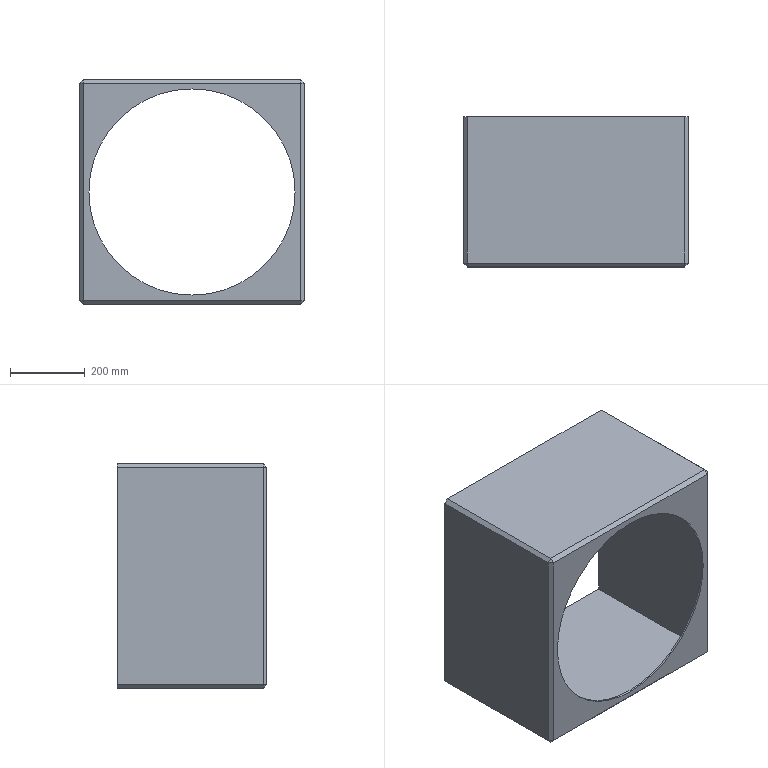Component | SolidWorks | Housing-1 | 1 solid | 25 faces | box 600 x 400 x 600 mm | volume 18742752 mm3 | plane 23 | cylinder 2 | commonest cylinder face diameters 550 x2
build123d program:
from build123d import *

# Parameters (mm, degrees)
SKETCH1_W           = 600
SKETCH1_H           = 600
SKETCH1_W_2         = 560
SKETCH1_H_2         = 560
BOSS_EXTRUDE1_DEPTH = 400
SKETCH2_W           = 560
SKETCH2_H           = 560
SKETCH2_R           = 275
BOSS_EXTRUDE2_DEPTH = 5
CHAMFER3_SIZE       = 10


with BuildPart() as part:
    # Sketch1 → Boss-Extrude1 (new body)
    with BuildSketch(Plane.XY):
        with Locations((-0.7059, 193.51)):
            Rectangle(SKETCH1_W, SKETCH1_H)
        with Locations((-0.7059, 193.51)):
            Rectangle(SKETCH1_W_2, SKETCH1_H_2, mode=Mode.SUBTRACT)
    extrude(amount=BOSS_EXTRUDE1_DEPTH)

    # Sketch2 → Boss-Extrude2 (add)
    with BuildSketch(Plane.XY.offset(400)):
        with Locations((-0.7059, 193.51)):
            Rectangle(SKETCH2_W, SKETCH2_H)
        with Locations((-0.7059, 193.51)):
            Circle(SKETCH2_R, mode=Mode.SUBTRACT)
    extrude(amount=-BOSS_EXTRUDE2_DEPTH)

    # Chamfer3
    chamfer3_edges = [part.edges().sort_by_distance(p)[0] for p in [
        (299.294, 193.51, 400),
        (-0.7059, 493.51, 400),
        (-300.706, 193.51, 400),
        (-300.706, 493.51, 200),
        (299.294, 493.51, 200),
        (299.294, -106.49, 200),
        (-300.706, -106.49, 200),
        (-0.7059, -106.49, 400),
    ]]
    chamfer(chamfer3_edges, length=CHAMFER3_SIZE)


solid = part.part

# Placed as in the assembly
solid = solid.moved(Location((0.7059, -200, -493.51), (90, 0, 0)))
STEP:
#1=COLOUR_RGB('',0.7922,0.8196,0.9333);
#2=FILL_AREA_STYLE_COLOUR('',#1);
#3=FILL_AREA_STYLE('',(#2));
#4=SURFACE_STYLE_FILL_AREA(#3);
#5=SURFACE_SIDE_STYLE('',(#4));
#6=SURFACE_STYLE_USAGE(.BOTH.,#5);
#7=PRESENTATION_STYLE_ASSIGNMENT((#6));
#8=CARTESIAN_POINT('',(10.827,-23.425,-11.811));
#9=VERTEX_POINT('',#8);
#10=CARTESIAN_POINT('',(-10.827,-23.425,-11.811));
#11=VERTEX_POINT('',#10);
#12=CARTESIAN_POINT('',(0.,-23.425,-11.811));
#13=DIRECTION('',(0.,-1.,0.));
#14=DIRECTION('',(-1.,0.,0.));
#15=AXIS2_PLACEMENT_3D('',#12,#13,#14);
#16=CIRCLE('',#15,10.827);
#17=EDGE_CURVE('',#9,#11,#16,.T.);
#18=ORIENTED_EDGE('',*,*,#17,.F.);
#19=CARTESIAN_POINT('',(10.827,-23.622,-11.811));
#20=VERTEX_POINT('',#19);
#21=CARTESIAN_POINT('',(10.827,-23.425,-11.811));
#22=DIRECTION('',(0.,-1.,0.));
#23=VECTOR('',#22,39.37);
#24=LINE('',#21,#23);
#25=EDGE_CURVE('',#9,#20,#24,.T.);
#26=ORIENTED_EDGE('',*,*,#25,.T.);
#27=CARTESIAN_POINT('',(-10.827,-23.622,-11.811));
#28=VERTEX_POINT('',#27);
#29=CARTESIAN_POINT('',(0.,-23.622,-11.811));
#30=DIRECTION('',(0.,-1.,0.));
#31=DIRECTION('',(-1.,0.,0.));
#32=AXIS2_PLACEMENT_3D('',#29,#30,#31);
#33=CIRCLE('',#32,10.827);
#34=EDGE_CURVE('',#20,#28,#33,.T.);
#35=ORIENTED_EDGE('',*,*,#34,.T.);
#36=CARTESIAN_POINT('',(-10.827,-23.425,-11.811));
#37=DIRECTION('',(0.,-1.,0.));
#38=VECTOR('',#37,39.37);
#39=LINE('',#36,#38);
#40=EDGE_CURVE('',#11,#28,#39,.T.);
#41=ORIENTED_EDGE('',*,*,#40,.F.);
#42=EDGE_LOOP('',(#18,#26,#35,#41));
#43=FACE_OUTER_BOUND('',#42,.T.);
#44=CARTESIAN_POINT('',(0.,-23.425,-11.811));
#45=DIRECTION('',(0.,-1.,0.));
#46=DIRECTION('',(-1.,0.,0.));
#47=AXIS2_PLACEMENT_3D('',#44,#45,#46);
#48=CYLINDRICAL_SURFACE('',#47,10.827);
#49=ADVANCED_FACE('',(#43),#48,.F.);
#50=CARTESIAN_POINT('',(11.024,-23.425,-22.835));
#51=VERTEX_POINT('',#50);
#52=CARTESIAN_POINT('',(11.024,-7.874,-22.835));
#53=VERTEX_POINT('',#52);
#54=CARTESIAN_POINT('',(11.024,-23.622,-22.835));
#55=DIRECTION('',(0.,1.,0.));
#56=VECTOR('',#55,39.37);
#57=LINE('',#54,#56);
#58=EDGE_CURVE('',#51,#53,#57,.T.);
#59=ORIENTED_EDGE('',*,*,#58,.F.);
#60=CARTESIAN_POINT('',(11.024,-23.425,-0.7874));
#61=VERTEX_POINT('',#60);
#62=CARTESIAN_POINT('',(11.024,-23.425,-0.7874));
#63=DIRECTION('',(0.,0.,1.));
#64=VECTOR('',#63,39.37);
#65=LINE('',#62,#64);
#66=EDGE_CURVE('',#51,#61,#65,.T.);
#67=ORIENTED_EDGE('',*,*,#66,.T.);
#68=CARTESIAN_POINT('',(11.024,-7.874,-0.7874));
#69=VERTEX_POINT('',#68);
#70=CARTESIAN_POINT('',(11.024,-23.622,-0.7874));
#71=DIRECTION('',(0.,1.,0.));
#72=VECTOR('',#71,39.37);
#73=LINE('',#70,#72);
#74=EDGE_CURVE('',#61,#69,#73,.T.);
#75=ORIENTED_EDGE('',*,*,#74,.T.);
#76=CARTESIAN_POINT('',(11.024,-7.874,-22.835));
#77=DIRECTION('',(0.,0.,1.));
#78=VECTOR('',#77,39.37);
#79=LINE('',#76,#78);
#80=EDGE_CURVE('',#53,#69,#79,.T.);
#81=ORIENTED_EDGE('',*,*,#80,.F.);
#82=EDGE_LOOP('',(#59,#67,#75,#81));
#83=FACE_OUTER_BOUND('',#82,.T.);
#84=CARTESIAN_POINT('',(11.024,-23.622,-22.835));
#85=DIRECTION('',(-1.,0.,0.));
#86=DIRECTION('',(0.,1.,0.));
#87=AXIS2_PLACEMENT_3D('',#84,#85,#86);
#88=PLANE('',#87);
#89=ADVANCED_FACE('',(#83),#88,.T.);
#90=ORIENTED_EDGE('',*,*,#74,.F.);
#91=CARTESIAN_POINT('',(-11.024,-23.425,-0.7874));
#92=VERTEX_POINT('',#91);
#93=CARTESIAN_POINT('',(-11.024,-23.425,-0.7874));
#94=DIRECTION('',(-1.,0.,0.));
#95=VECTOR('',#94,39.37);
#96=LINE('',#93,#95);
#97=EDGE_CURVE('',#61,#92,#96,.T.);
#98=ORIENTED_EDGE('',*,*,#97,.T.);
#99=CARTESIAN_POINT('',(-11.024,-7.874,-0.7874));
#100=VERTEX_POINT('',#99);
#101=CARTESIAN_POINT('',(-11.024,-23.622,-0.7874));
#102=DIRECTION('',(0.,1.,0.));
#103=VECTOR('',#102,39.37);
#104=LINE('',#101,#103);
#105=EDGE_CURVE('',#92,#100,#104,.T.);
#106=ORIENTED_EDGE('',*,*,#105,.T.);
#107=CARTESIAN_POINT('',(11.024,-7.874,-0.7874));
#108=DIRECTION('',(-1.,0.,0.));
#109=VECTOR('',#108,39.37);
#110=LINE('',#107,#109);
#111=EDGE_CURVE('',#69,#100,#110,.T.);
#112=ORIENTED_EDGE('',*,*,#111,.F.);
#113=EDGE_LOOP('',(#90,#98,#106,#112));
#114=FACE_OUTER_BOUND('',#113,.T.);
#115=CARTESIAN_POINT('',(11.024,-23.622,-0.7874));
#116=DIRECTION('',(-0.,0.,-1.));
#117=DIRECTION('',(1.,0.,-0.));
#118=AXIS2_PLACEMENT_3D('',#115,#116,#117);
#119=PLANE('',#118);
#120=ADVANCED_FACE('',(#114),#119,.T.);
#121=ORIENTED_EDGE('',*,*,#105,.F.);
#122=CARTESIAN_POINT('',(-11.024,-23.425,-22.835));
#123=VERTEX_POINT('',#122);
#124=CARTESIAN_POINT('',(-11.024,-23.425,-0.7874));
#125=DIRECTION('',(0.,0.,-1.));
#126=VECTOR('',#125,39.37);
#127=LINE('',#124,#126);
#128=EDGE_CURVE('',#92,#123,#127,.T.);
#129=ORIENTED_EDGE('',*,*,#128,.T.);
#130=CARTESIAN_POINT('',(-11.024,-7.874,-22.835));
#131=VERTEX_POINT('',#130);
#132=CARTESIAN_POINT('',(-11.024,-23.622,-22.835));
#133=DIRECTION('',(0.,1.,0.));
#134=VECTOR('',#133,39.37);
#135=LINE('',#132,#134);
#136=EDGE_CURVE('',#123,#131,#135,.T.);
#137=ORIENTED_EDGE('',*,*,#136,.T.);
#138=CARTESIAN_POINT('',(-11.024,-7.874,-22.835));
#139=DIRECTION('',(0.,0.,-1.));
#140=VECTOR('',#139,39.37);
#141=LINE('',#138,#140);
#142=EDGE_CURVE('',#100,#131,#141,.T.);
#143=ORIENTED_EDGE('',*,*,#142,.F.);
#144=EDGE_LOOP('',(#121,#129,#137,#143));
#145=FACE_OUTER_BOUND('',#144,.T.);
#146=CARTESIAN_POINT('',(-11.024,-23.622,-22.835));
#147=DIRECTION('',(1.,0.,0.));
#148=DIRECTION('',(0.,-1.,0.));
#149=AXIS2_PLACEMENT_3D('',#146,#147,#148);
#150=PLANE('',#149);
#151=ADVANCED_FACE('',(#145),#150,.T.);
#152=ORIENTED_EDGE('',*,*,#136,.F.);
#153=CARTESIAN_POINT('',(-11.024,-23.425,-22.835));
#154=DIRECTION('',(1.,0.,0.));
#155=VECTOR('',#154,39.37);
#156=LINE('',#153,#155);
#157=EDGE_CURVE('',#123,#51,#156,.T.);
#158=ORIENTED_EDGE('',*,*,#157,.T.);
#159=ORIENTED_EDGE('',*,*,#58,.T.);
#160=CARTESIAN_POINT('',(11.024,-7.874,-22.835));
#161=DIRECTION('',(1.,0.,0.));
#162=VECTOR('',#161,39.37);
#163=LINE('',#160,#162);
#164=EDGE_CURVE('',#131,#53,#163,.T.);
#165=ORIENTED_EDGE('',*,*,#164,.F.);
#166=EDGE_LOOP('',(#152,#158,#159,#165));
#167=FACE_OUTER_BOUND('',#166,.T.);
#168=CARTESIAN_POINT('',(11.024,-23.622,-22.835));
#169=DIRECTION('',(0.,0.,1.));
#170=DIRECTION('',(0.,1.,0.));
#171=AXIS2_PLACEMENT_3D('',#168,#169,#170);
#172=PLANE('',#171);
#173=ADVANCED_FACE('',(#167),#172,.T.);
#174=CARTESIAN_POINT('',(-11.417,-23.622,-23.228));
#175=VERTEX_POINT('',#174);
#176=CARTESIAN_POINT('',(11.417,-23.622,-23.228));
#177=VERTEX_POINT('',#176);
#178=CARTESIAN_POINT('',(11.811,-23.622,-23.228));
#179=DIRECTION('',(1.,0.,0.));
#180=VECTOR('',#179,39.37);
#181=LINE('',#178,#180);
#182=EDGE_CURVE('',#175,#177,#181,.T.);
#183=ORIENTED_EDGE('',*,*,#182,.T.);
#184=CARTESIAN_POINT('',(11.417,-23.622,-0.3937));
#185=VERTEX_POINT('',#184);
#186=CARTESIAN_POINT('',(11.417,-23.622,0.));
#187=DIRECTION('',(-0.,0.,1.));
#188=VECTOR('',#187,39.37);
#189=LINE('',#186,#188);
#190=EDGE_CURVE('',#177,#185,#189,.T.);
#191=ORIENTED_EDGE('',*,*,#190,.T.);
#192=CARTESIAN_POINT('',(-11.417,-23.622,-0.3937));
#193=VERTEX_POINT('',#192);
#194=CARTESIAN_POINT('',(-11.811,-23.622,-0.3937));
#195=DIRECTION('',(-1.,0.,0.));
#196=VECTOR('',#195,39.37);
#197=LINE('',#194,#196);
#198=EDGE_CURVE('',#185,#193,#197,.T.);
#199=ORIENTED_EDGE('',*,*,#198,.T.);
#200=CARTESIAN_POINT('',(-11.417,-23.622,-23.622));
#201=DIRECTION('',(0.,0.,-1.));
#202=VECTOR('',#201,39.37);
#203=LINE('',#200,#202);
#204=EDGE_CURVE('',#193,#175,#203,.T.);
#205=ORIENTED_EDGE('',*,*,#204,.T.);
#206=EDGE_LOOP('',(#183,#191,#199,#205));
#207=FACE_OUTER_BOUND('',#206,.T.);
#208=CARTESIAN_POINT('',(0.,-23.622,-11.811));
#209=DIRECTION('',(0.,-1.,0.));
#210=DIRECTION('',(-1.,0.,0.));
#211=AXIS2_PLACEMENT_3D('',#208,#209,#210);
#212=CIRCLE('',#211,10.827);
#213=EDGE_CURVE('',#28,#20,#212,.T.);
#214=ORIENTED_EDGE('',*,*,#213,.F.);
#215=ORIENTED_EDGE('',*,*,#34,.F.);
#216=EDGE_LOOP('',(#214,#215));
#217=FACE_BOUND('',#216,.T.);
#218=CARTESIAN_POINT('',(-0.02779,-23.622,-4.193));
#219=DIRECTION('',(0.,-1.,0.));
#220=DIRECTION('',(-1.,0.,0.));
#221=AXIS2_PLACEMENT_3D('',#218,#219,#220);
#222=PLANE('',#221);
#223=ADVANCED_FACE('',(#207,#217),#222,.T.);
#224=CARTESIAN_POINT('',(11.811,-7.874,-23.228));
#225=VERTEX_POINT('',#224);
#226=CARTESIAN_POINT('',(11.811,-7.874,-0.3937));
#227=VERTEX_POINT('',#226);
#228=CARTESIAN_POINT('',(11.811,-7.874,-23.622));
#229=DIRECTION('',(-0.,0.,1.));
#230=VECTOR('',#229,39.37);
#231=LINE('',#228,#230);
#232=EDGE_CURVE('',#225,#227,#231,.T.);
#233=ORIENTED_EDGE('',*,*,#232,.F.);
#234=CARTESIAN_POINT('',(11.417,-7.874,-23.622));
#235=VERTEX_POINT('',#234);
#236=CARTESIAN_POINT('',(11.811,-7.874,-23.228));
#237=DIRECTION('',(-0.7071,0.,-0.7071));
#238=VECTOR('',#237,39.37);
#239=LINE('',#236,#238);
#240=EDGE_CURVE('',#225,#235,#239,.T.);
#241=ORIENTED_EDGE('',*,*,#240,.T.);
#242=CARTESIAN_POINT('',(-11.417,-7.874,-23.622));
#243=VERTEX_POINT('',#242);
#244=CARTESIAN_POINT('',(11.811,-7.874,-23.622));
#245=DIRECTION('',(1.,0.,0.));
#246=VECTOR('',#245,39.37);
#247=LINE('',#244,#246);
#248=EDGE_CURVE('',#243,#235,#247,.T.);
#249=ORIENTED_EDGE('',*,*,#248,.F.);
#250=CARTESIAN_POINT('',(-11.811,-7.874,-23.228));
#251=VERTEX_POINT('',#250);
#252=CARTESIAN_POINT('',(-11.417,-7.874,-23.622));
#253=DIRECTION('',(-0.7071,0.,0.7071));
#254=VECTOR('',#253,39.37);
#255=LINE('',#252,#254);
#256=EDGE_CURVE('',#243,#251,#255,.T.);
#257=ORIENTED_EDGE('',*,*,#256,.T.);
#258=CARTESIAN_POINT('',(-11.811,-7.874,-0.3937));
#259=VERTEX_POINT('',#258);
#260=CARTESIAN_POINT('',(-11.811,-7.874,-23.622));
#261=DIRECTION('',(0.,0.,-1.));
#262=VECTOR('',#261,39.37);
#263=LINE('',#260,#262);
#264=EDGE_CURVE('',#259,#251,#263,.T.);
#265=ORIENTED_EDGE('',*,*,#264,.F.);
#266=CARTESIAN_POINT('',(-11.417,-7.874,0.));
#267=VERTEX_POINT('',#266);
#268=CARTESIAN_POINT('',(-11.811,-7.874,-0.3937));
#269=DIRECTION('',(0.7071,0.,0.7071));
#270=VECTOR('',#269,39.37);
#271=LINE('',#268,#270);
#272=EDGE_CURVE('',#259,#267,#271,.T.);
#273=ORIENTED_EDGE('',*,*,#272,.T.);
#274=CARTESIAN_POINT('',(11.417,-7.874,0.));
#275=VERTEX_POINT('',#274);
#276=CARTESIAN_POINT('',(11.811,-7.874,0.));
#277=DIRECTION('',(-1.,0.,0.));
#278=VECTOR('',#277,39.37);
#279=LINE('',#276,#278);
#280=EDGE_CURVE('',#275,#267,#279,.T.);
#281=ORIENTED_EDGE('',*,*,#280,.F.);
#282=CARTESIAN_POINT('',(11.417,-7.874,0.));
#283=DIRECTION('',(0.7071,0.,-0.7071));
#284=VECTOR('',#283,39.37);
#285=LINE('',#282,#284);
#286=EDGE_CURVE('',#275,#227,#285,.T.);
#287=ORIENTED_EDGE('',*,*,#286,.T.);
#288=EDGE_LOOP('',(#233,#241,#249,#257,#265,#273,#281,#287));
#289=FACE_OUTER_BOUND('',#288,.T.);
#290=ORIENTED_EDGE('',*,*,#80,.T.);
#291=ORIENTED_EDGE('',*,*,#111,.T.);
#292=ORIENTED_EDGE('',*,*,#142,.T.);
#293=ORIENTED_EDGE('',*,*,#164,.T.);
#294=EDGE_LOOP('',(#290,#291,#292,#293));
#295=FACE_BOUND('',#294,.T.);
#296=CARTESIAN_POINT('',(-0.02779,-7.874,-4.193));
#297=DIRECTION('',(0.,-1.,0.));
#298=DIRECTION('',(-1.,0.,0.));
#299=AXIS2_PLACEMENT_3D('',#296,#297,#298);
#300=PLANE('',#299);
#301=ADVANCED_FACE('',(#289,#295),#300,.F.);
#302=CARTESIAN_POINT('',(11.811,-23.228,-0.3937));
#303=VERTEX_POINT('',#302);
#304=CARTESIAN_POINT('',(11.811,-23.228,-23.228));
#305=VERTEX_POINT('',#304);
#306=CARTESIAN_POINT('',(11.811,-23.228,-23.622));
#307=DIRECTION('',(0.,0.,-1.));
#308=VECTOR('',#307,39.37);
#309=LINE('',#306,#308);
#310=EDGE_CURVE('',#303,#305,#309,.T.);
#311=ORIENTED_EDGE('',*,*,#310,.T.);
#312=CARTESIAN_POINT('',(11.811,-23.622,-23.228));
#313=DIRECTION('',(0.,1.,0.));
#314=VECTOR('',#313,39.37);
#315=LINE('',#312,#314);
#316=EDGE_CURVE('',#305,#225,#315,.T.);
#317=ORIENTED_EDGE('',*,*,#316,.T.);
#318=ORIENTED_EDGE('',*,*,#232,.T.);
#319=CARTESIAN_POINT('',(11.811,-23.622,-0.3937));
#320=DIRECTION('',(0.,-1.,0.));
#321=VECTOR('',#320,39.37);
#322=LINE('',#319,#321);
#323=EDGE_CURVE('',#227,#303,#322,.T.);
#324=ORIENTED_EDGE('',*,*,#323,.T.);
#325=EDGE_LOOP('',(#311,#317,#318,#324));
#326=FACE_OUTER_BOUND('',#325,.T.);
#327=CARTESIAN_POINT('',(11.811,-23.622,-23.622));
#328=DIRECTION('',(-1.,0.,-0.));
#329=DIRECTION('',(0.,0.,-1.));
#330=AXIS2_PLACEMENT_3D('',#327,#328,#329);
#331=PLANE('',#330);
#332=ADVANCED_FACE('',(#326),#331,.F.);
#333=CARTESIAN_POINT('',(-11.417,-23.228,0.));
#334=VERTEX_POINT('',#333);
#335=CARTESIAN_POINT('',(11.417,-23.228,0.));
#336=VERTEX_POINT('',#335);
#337=CARTESIAN_POINT('',(11.811,-23.228,0.));
#338=DIRECTION('',(1.,0.,0.));
#339=VECTOR('',#338,39.37);
#340=LINE('',#337,#339);
#341=EDGE_CURVE('',#334,#336,#340,.T.);
#342=ORIENTED_EDGE('',*,*,#341,.T.);
#343=CARTESIAN_POINT('',(11.417,-23.622,0.));
#344=DIRECTION('',(0.,1.,0.));
#345=VECTOR('',#344,39.37);
#346=LINE('',#343,#345);
#347=EDGE_CURVE('',#336,#275,#346,.T.);
#348=ORIENTED_EDGE('',*,*,#347,.T.);
#349=ORIENTED_EDGE('',*,*,#280,.T.);
#350=CARTESIAN_POINT('',(-11.417,-23.622,0.));
#351=DIRECTION('',(0.,-1.,0.));
#352=VECTOR('',#351,39.37);
#353=LINE('',#350,#352);
#354=EDGE_CURVE('',#267,#334,#353,.T.);
#355=ORIENTED_EDGE('',*,*,#354,.T.);
#356=EDGE_LOOP('',(#342,#348,#349,#355));
#357=FACE_OUTER_BOUND('',#356,.T.);
#358=CARTESIAN_POINT('',(11.811,-23.622,0.));
#359=DIRECTION('',(0.,0.,-1.));
#360=DIRECTION('',(0.,-1.,0.));
#361=AXIS2_PLACEMENT_3D('',#358,#359,#360);
#362=PLANE('',#361);
#363=ADVANCED_FACE('',(#357),#362,.F.);
#364=CARTESIAN_POINT('',(-11.811,-23.228,-23.228));
#365=VERTEX_POINT('',#364);
#366=CARTESIAN_POINT('',(-11.811,-23.228,-0.3937));
#367=VERTEX_POINT('',#366);
#368=CARTESIAN_POINT('',(-11.811,-23.228,0.));
#369=DIRECTION('',(-0.,0.,1.));
#370=VECTOR('',#369,39.37);
#371=LINE('',#368,#370);
#372=EDGE_CURVE('',#365,#367,#371,.T.);
#373=ORIENTED_EDGE('',*,*,#372,.T.);
#374=CARTESIAN_POINT('',(-11.811,-23.622,-0.3937));
#375=DIRECTION('',(0.,1.,0.));
#376=VECTOR('',#375,39.37);
#377=LINE('',#374,#376);
#378=EDGE_CURVE('',#367,#259,#377,.T.);
#379=ORIENTED_EDGE('',*,*,#378,.T.);
#380=ORIENTED_EDGE('',*,*,#264,.T.);
#381=CARTESIAN_POINT('',(-11.811,-23.622,-23.228));
#382=DIRECTION('',(0.,-1.,0.));
#383=VECTOR('',#382,39.37);
#384=LINE('',#381,#383);
#385=EDGE_CURVE('',#251,#365,#384,.T.);
#386=ORIENTED_EDGE('',*,*,#385,.T.);
#387=EDGE_LOOP('',(#373,#379,#380,#386));
#388=FACE_OUTER_BOUND('',#387,.T.);
#389=CARTESIAN_POINT('',(-11.811,-23.622,-23.622));
#390=DIRECTION('',(1.,0.,0.));
#391=DIRECTION('',(-0.,0.,1.));
#392=AXIS2_PLACEMENT_3D('',#389,#390,#391);
#393=PLANE('',#392);
#394=ADVANCED_FACE('',(#388),#393,.F.);
#395=ORIENTED_EDGE('',*,*,#248,.T.);
#396=CARTESIAN_POINT('',(11.417,-23.228,-23.622));
#397=VERTEX_POINT('',#396);
#398=CARTESIAN_POINT('',(11.417,-23.622,-23.622));
#399=DIRECTION('',(0.,-1.,0.));
#400=VECTOR('',#399,39.37);
#401=LINE('',#398,#400);
#402=EDGE_CURVE('',#235,#397,#401,.T.);
#403=ORIENTED_EDGE('',*,*,#402,.T.);
#404=CARTESIAN_POINT('',(-11.417,-23.228,-23.622));
#405=VERTEX_POINT('',#404);
#406=CARTESIAN_POINT('',(-11.811,-23.228,-23.622));
#407=DIRECTION('',(-1.,0.,0.));
#408=VECTOR('',#407,39.37);
#409=LINE('',#406,#408);
#410=EDGE_CURVE('',#397,#405,#409,.T.);
#411=ORIENTED_EDGE('',*,*,#410,.T.);
#412=CARTESIAN_POINT('',(-11.417,-23.622,-23.622));
#413=DIRECTION('',(0.,1.,0.));
#414=VECTOR('',#413,39.37);
#415=LINE('',#412,#414);
#416=EDGE_CURVE('',#405,#243,#415,.T.);
#417=ORIENTED_EDGE('',*,*,#416,.T.);
#418=EDGE_LOOP('',(#395,#403,#411,#417));
#419=FACE_OUTER_BOUND('',#418,.T.);
#420=CARTESIAN_POINT('',(11.811,-23.622,-23.622));
#421=DIRECTION('',(0.,0.,1.));
#422=DIRECTION('',(0.,1.,0.));
#423=AXIS2_PLACEMENT_3D('',#420,#421,#422);
#424=PLANE('',#423);
#425=ADVANCED_FACE('',(#419),#424,.F.);
#426=CARTESIAN_POINT('',(0.,-23.425,-11.811));
#427=DIRECTION('',(0.,-1.,0.));
#428=DIRECTION('',(-1.,0.,0.));
#429=AXIS2_PLACEMENT_3D('',#426,#427,#428);
#430=CIRCLE('',#429,10.827);
#431=EDGE_CURVE('',#11,#9,#430,.T.);
#432=ORIENTED_EDGE('',*,*,#431,.T.);
#433=ORIENTED_EDGE('',*,*,#17,.T.);
#434=EDGE_LOOP('',(#432,#433));
#435=FACE_BOUND('',#434,.T.);
#436=ORIENTED_EDGE('',*,*,#128,.F.);
#437=ORIENTED_EDGE('',*,*,#97,.F.);
#438=ORIENTED_EDGE('',*,*,#66,.F.);
#439=ORIENTED_EDGE('',*,*,#157,.F.);
#440=EDGE_LOOP('',(#436,#437,#438,#439));
#441=FACE_OUTER_BOUND('',#440,.T.);
#442=CARTESIAN_POINT('',(-0.02779,-23.425,-4.193));
#443=DIRECTION('',(0.,-1.,0.));
#444=DIRECTION('',(-1.,0.,0.));
#445=AXIS2_PLACEMENT_3D('',#442,#443,#444);
#446=PLANE('',#445);
#447=ADVANCED_FACE('',(#435,#441),#446,.F.);
#448=ORIENTED_EDGE('',*,*,#25,.F.);
#449=ORIENTED_EDGE('',*,*,#431,.F.);
#450=ORIENTED_EDGE('',*,*,#40,.T.);
#451=ORIENTED_EDGE('',*,*,#213,.T.);
#452=EDGE_LOOP('',(#448,#449,#450,#451));
#453=FACE_OUTER_BOUND('',#452,.T.);
#454=CARTESIAN_POINT('',(0.,-23.425,-11.811));
#455=DIRECTION('',(0.,-1.,0.));
#456=DIRECTION('',(-1.,0.,0.));
#457=AXIS2_PLACEMENT_3D('',#454,#455,#456);
#458=CYLINDRICAL_SURFACE('',#457,10.827);
#459=ADVANCED_FACE('',(#453),#458,.F.);
#460=ORIENTED_EDGE('',*,*,#256,.F.);
#461=ORIENTED_EDGE('',*,*,#416,.F.);
#462=CARTESIAN_POINT('',(-11.417,-23.228,-23.622));
#463=DIRECTION('',(0.7071,-0.,-0.7071));
#464=VECTOR('',#463,39.37);
#465=LINE('',#462,#464);
#466=EDGE_CURVE('',#365,#405,#465,.T.);
#467=ORIENTED_EDGE('',*,*,#466,.F.);
#468=ORIENTED_EDGE('',*,*,#385,.F.);
#469=EDGE_LOOP('',(#460,#461,#467,#468));
#470=FACE_OUTER_BOUND('',#469,.T.);
#471=CARTESIAN_POINT('',(-11.417,-23.622,-23.622));
#472=DIRECTION('',(0.7071,0.,0.7071));
#473=DIRECTION('',(0.,1.,0.));
#474=AXIS2_PLACEMENT_3D('',#471,#472,#473);
#475=PLANE('',#474);
#476=ADVANCED_FACE('',(#470),#475,.F.);
#477=CARTESIAN_POINT('',(-11.417,-23.622,-0.3937));
#478=DIRECTION('',(0.7071,-0.7071,0.));
#479=VECTOR('',#478,39.37);
#480=LINE('',#477,#479);
#481=EDGE_CURVE('',#367,#193,#480,.T.);
#482=ORIENTED_EDGE('',*,*,#481,.F.);
#483=ORIENTED_EDGE('',*,*,#372,.F.);
#484=CARTESIAN_POINT('',(-11.614,-23.425,-23.228));
#485=DIRECTION('',(-0.7071,0.7071,-0.));
#486=VECTOR('',#485,39.37);
#487=LINE('',#484,#486);
#488=EDGE_CURVE('',#175,#365,#487,.T.);
#489=ORIENTED_EDGE('',*,*,#488,.F.);
#490=ORIENTED_EDGE('',*,*,#204,.F.);
#491=EDGE_LOOP('',(#482,#483,#489,#490));
#492=FACE_OUTER_BOUND('',#491,.T.);
#493=CARTESIAN_POINT('',(-11.417,-23.622,-4.193));
#494=DIRECTION('',(-0.7071,-0.7071,-0.));
#495=DIRECTION('',(-0.,0.,1.));
#496=AXIS2_PLACEMENT_3D('',#493,#494,#495);
#497=PLANE('',#496);
#498=ADVANCED_FACE('',(#492),#497,.T.);
#499=ORIENTED_EDGE('',*,*,#272,.F.);
#500=ORIENTED_EDGE('',*,*,#378,.F.);
#501=CARTESIAN_POINT('',(-11.614,-23.228,-0.1969));
#502=DIRECTION('',(-0.7071,0.,-0.7071));
#503=VECTOR('',#502,39.37);
#504=LINE('',#501,#503);
#505=EDGE_CURVE('',#334,#367,#504,.T.);
#506=ORIENTED_EDGE('',*,*,#505,.F.);
#507=ORIENTED_EDGE('',*,*,#354,.F.);
#508=EDGE_LOOP('',(#499,#500,#506,#507));
#509=FACE_OUTER_BOUND('',#508,.T.);
#510=CARTESIAN_POINT('',(-11.811,-23.622,-0.3937));
#511=DIRECTION('',(0.7071,0.,-0.7071));
#512=DIRECTION('',(0.,1.,0.));
#513=AXIS2_PLACEMENT_3D('',#510,#511,#512);
#514=PLANE('',#513);
#515=ADVANCED_FACE('',(#509),#514,.F.);
#516=ORIENTED_EDGE('',*,*,#488,.T.);
#517=ORIENTED_EDGE('',*,*,#466,.T.);
#518=CARTESIAN_POINT('',(-11.417,-23.228,-23.622));
#519=DIRECTION('',(0.,0.7071,-0.7071));
#520=VECTOR('',#519,39.37);
#521=LINE('',#518,#520);
#522=EDGE_CURVE('',#175,#405,#521,.T.);
#523=ORIENTED_EDGE('',*,*,#522,.F.);
#524=EDGE_LOOP('',(#516,#517,#523));
#525=FACE_OUTER_BOUND('',#524,.T.);
#526=CARTESIAN_POINT('',(-11.417,-23.228,-23.622));
#527=DIRECTION('',(-0.5774,-0.5774,-0.5774));
#528=DIRECTION('',(-0.7071,0.7071,0.));
#529=AXIS2_PLACEMENT_3D('',#526,#527,#528);
#530=PLANE('',#529);
#531=ADVANCED_FACE('',(#525),#530,.T.);
#532=ORIENTED_EDGE('',*,*,#505,.T.);
#533=ORIENTED_EDGE('',*,*,#481,.T.);
#534=CARTESIAN_POINT('',(-11.417,-23.622,-0.3937));
#535=DIRECTION('',(-0.,-0.7071,-0.7071));
#536=VECTOR('',#535,39.37);
#537=LINE('',#534,#536);
#538=EDGE_CURVE('',#334,#193,#537,.T.);
#539=ORIENTED_EDGE('',*,*,#538,.F.);
#540=EDGE_LOOP('',(#532,#533,#539));
#541=FACE_OUTER_BOUND('',#540,.T.);
#542=CARTESIAN_POINT('',(-11.417,-23.622,-0.3937));
#543=DIRECTION('',(-0.5774,-0.5774,0.5774));
#544=DIRECTION('',(-0.7071,0.,-0.7071));
#545=AXIS2_PLACEMENT_3D('',#542,#543,#544);
#546=PLANE('',#545);
#547=ADVANCED_FACE('',(#541),#546,.T.);
#548=ORIENTED_EDGE('',*,*,#240,.F.);
#549=ORIENTED_EDGE('',*,*,#316,.F.);
#550=CARTESIAN_POINT('',(11.811,-23.228,-23.228));
#551=DIRECTION('',(0.7071,0.,0.7071));
#552=VECTOR('',#551,39.37);
#553=LINE('',#550,#552);
#554=EDGE_CURVE('',#397,#305,#553,.T.);
#555=ORIENTED_EDGE('',*,*,#554,.F.);
#556=ORIENTED_EDGE('',*,*,#402,.F.);
#557=EDGE_LOOP('',(#548,#549,#555,#556));
#558=FACE_OUTER_BOUND('',#557,.T.);
#559=CARTESIAN_POINT('',(11.811,-23.622,-23.228));
#560=DIRECTION('',(-0.7071,0.,0.7071));
#561=DIRECTION('',(0.,1.,0.));
#562=AXIS2_PLACEMENT_3D('',#559,#560,#561);
#563=PLANE('',#562);
#564=ADVANCED_FACE('',(#558),#563,.F.);
#565=ORIENTED_EDGE('',*,*,#522,.T.);
#566=ORIENTED_EDGE('',*,*,#410,.F.);
#567=CARTESIAN_POINT('',(11.417,-23.425,-23.425));
#568=DIRECTION('',(0.,0.7071,-0.7071));
#569=VECTOR('',#568,39.37);
#570=LINE('',#567,#569);
#571=EDGE_CURVE('',#177,#397,#570,.T.);
#572=ORIENTED_EDGE('',*,*,#571,.F.);
#573=ORIENTED_EDGE('',*,*,#182,.F.);
#574=EDGE_LOOP('',(#565,#566,#572,#573));
#575=FACE_OUTER_BOUND('',#574,.T.);
#576=CARTESIAN_POINT('',(-0.02779,-23.622,-23.228));
#577=DIRECTION('',(0.,-0.7071,-0.7071));
#578=DIRECTION('',(-1.,0.,0.));
#579=AXIS2_PLACEMENT_3D('',#576,#577,#578);
#580=PLANE('',#579);
#581=ADVANCED_FACE('',(#575),#580,.T.);
#582=ORIENTED_EDGE('',*,*,#538,.T.);
#583=ORIENTED_EDGE('',*,*,#198,.F.);
#584=CARTESIAN_POINT('',(11.417,-23.622,-0.3937));
#585=DIRECTION('',(-0.,-0.7071,-0.7071));
#586=VECTOR('',#585,39.37);
#587=LINE('',#584,#586);
#588=EDGE_CURVE('',#336,#185,#587,.T.);
#589=ORIENTED_EDGE('',*,*,#588,.F.);
#590=ORIENTED_EDGE('',*,*,#341,.F.);
#591=EDGE_LOOP('',(#582,#583,#589,#590));
#592=FACE_OUTER_BOUND('',#591,.T.);
#593=CARTESIAN_POINT('',(-0.02779,-23.622,-0.3937));
#594=DIRECTION('',(0.,-0.7071,0.7071));
#595=DIRECTION('',(1.,0.,0.));
#596=AXIS2_PLACEMENT_3D('',#593,#594,#595);
#597=PLANE('',#596);
#598=ADVANCED_FACE('',(#592),#597,.T.);
#599=ORIENTED_EDGE('',*,*,#286,.F.);
#600=ORIENTED_EDGE('',*,*,#347,.F.);
#601=CARTESIAN_POINT('',(11.614,-23.228,-0.1969));
#602=DIRECTION('',(-0.7071,0.,0.7071));
#603=VECTOR('',#602,39.37);
#604=LINE('',#601,#603);
#605=EDGE_CURVE('',#303,#336,#604,.T.);
#606=ORIENTED_EDGE('',*,*,#605,.F.);
#607=ORIENTED_EDGE('',*,*,#323,.F.);
#608=EDGE_LOOP('',(#599,#600,#606,#607));
#609=FACE_OUTER_BOUND('',#608,.T.);
#610=CARTESIAN_POINT('',(11.417,-23.622,0.));
#611=DIRECTION('',(-0.7071,0.,-0.7071));
#612=DIRECTION('',(0.,1.,0.));
#613=AXIS2_PLACEMENT_3D('',#610,#611,#612);
#614=PLANE('',#613);
#615=ADVANCED_FACE('',(#609),#614,.F.);
#616=ORIENTED_EDGE('',*,*,#571,.T.);
#617=ORIENTED_EDGE('',*,*,#554,.T.);
#618=CARTESIAN_POINT('',(11.811,-23.228,-23.228));
#619=DIRECTION('',(0.7071,0.7071,0.));
#620=VECTOR('',#619,39.37);
#621=LINE('',#618,#620);
#622=EDGE_CURVE('',#177,#305,#621,.T.);
#623=ORIENTED_EDGE('',*,*,#622,.F.);
#624=EDGE_LOOP('',(#616,#617,#623));
#625=FACE_OUTER_BOUND('',#624,.T.);
#626=CARTESIAN_POINT('',(11.811,-23.228,-23.228));
#627=DIRECTION('',(0.5774,-0.5774,-0.5774));
#628=DIRECTION('',(-0.7071,-0.7071,0.));
#629=AXIS2_PLACEMENT_3D('',#626,#627,#628);
#630=PLANE('',#629);
#631=ADVANCED_FACE('',(#625),#630,.T.);
#632=ORIENTED_EDGE('',*,*,#605,.T.);
#633=ORIENTED_EDGE('',*,*,#588,.T.);
#634=CARTESIAN_POINT('',(11.417,-23.622,-0.3937));
#635=DIRECTION('',(-0.7071,-0.7071,0.));
#636=VECTOR('',#635,39.37);
#637=LINE('',#634,#636);
#638=EDGE_CURVE('',#303,#185,#637,.T.);
#639=ORIENTED_EDGE('',*,*,#638,.F.);
#640=EDGE_LOOP('',(#632,#633,#639));
#641=FACE_OUTER_BOUND('',#640,.T.);
#642=CARTESIAN_POINT('',(11.417,-23.622,-0.3937));
#643=DIRECTION('',(0.5774,-0.5774,0.5774));
#644=DIRECTION('',(-0.7071,0.,0.7071));
#645=AXIS2_PLACEMENT_3D('',#642,#643,#644);
#646=PLANE('',#645);
#647=ADVANCED_FACE('',(#641),#646,.T.);
#648=ORIENTED_EDGE('',*,*,#622,.T.);
#649=ORIENTED_EDGE('',*,*,#310,.F.);
#650=ORIENTED_EDGE('',*,*,#638,.T.);
#651=ORIENTED_EDGE('',*,*,#190,.F.);
#652=EDGE_LOOP('',(#648,#649,#650,#651));
#653=FACE_OUTER_BOUND('',#652,.T.);
#654=CARTESIAN_POINT('',(11.417,-23.622,-4.193));
#655=DIRECTION('',(0.7071,-0.7071,0.));
#656=DIRECTION('',(0.,0.,-1.));
#657=AXIS2_PLACEMENT_3D('',#654,#655,#656);
#658=PLANE('',#657);
#659=ADVANCED_FACE('',(#653),#658,.T.);
#660=CLOSED_SHELL('',(#49,#89,#120,#151,#173,#223,#301,#332,#363,#394,#425,#447,#459,#476,#498,#515,#531,#547,#564,#581,#598,#615,#631,#647,#659));
#661=MANIFOLD_SOLID_BREP('',#660);
#662=STYLED_ITEM('',(#7),#661);
#663=(LENGTH_UNIT()NAMED_UNIT(*)SI_UNIT($,.METRE.));
#664=LENGTH_MEASURE_WITH_UNIT(LENGTH_MEASURE(0.0254),#663);
#665=DIMENSIONAL_EXPONENTS(1.,0.,0.,0.,0.,0.,0.);
#666=(CONVERSION_BASED_UNIT('',#664)LENGTH_UNIT()NAMED_UNIT(#665));
#667=UNCERTAINTY_MEASURE_WITH_UNIT(LENGTH_MEASURE(0.00001),#666,'','');
#668=(NAMED_UNIT(*)PLANE_ANGLE_UNIT()SI_UNIT($,.RADIAN.));
#669=(NAMED_UNIT(*)SI_UNIT($,.STERADIAN.)SOLID_ANGLE_UNIT());
#670=(GEOMETRIC_REPRESENTATION_CONTEXT(3)GLOBAL_UNCERTAINTY_ASSIGNED_CONTEXT((#667))GLOBAL_UNIT_ASSIGNED_CONTEXT((#666,#668,#669))REPRESENTATION_CONTEXT('',''));
#671=MECHANICAL_DESIGN_GEOMETRIC_PRESENTATION_REPRESENTATION('',(#662),#670);
#672=CARTESIAN_POINT('',(0.,0.,0.));
#673=DIRECTION('',(0.,0.,1.));
#674=DIRECTION('',(1.,0.,0.));
#675=AXIS2_PLACEMENT_3D('',#672,#673,#674);
#676=(LENGTH_UNIT()NAMED_UNIT(*)SI_UNIT($,.METRE.));
#677=LENGTH_MEASURE_WITH_UNIT(LENGTH_MEASURE(0.0254),#676);
#678=DIMENSIONAL_EXPONENTS(1.,0.,0.,0.,0.,0.,0.);
#679=(CONVERSION_BASED_UNIT('',#677)LENGTH_UNIT()NAMED_UNIT(#678));
#680=UNCERTAINTY_MEASURE_WITH_UNIT(LENGTH_MEASURE(0.00001),#679,'','');
#681=(NAMED_UNIT(*)PLANE_ANGLE_UNIT()SI_UNIT($,.RADIAN.));
#682=(NAMED_UNIT(*)SI_UNIT($,.STERADIAN.)SOLID_ANGLE_UNIT());
#683=(GEOMETRIC_REPRESENTATION_CONTEXT(3)GLOBAL_UNCERTAINTY_ASSIGNED_CONTEXT((#680))GLOBAL_UNIT_ASSIGNED_CONTEXT((#679,#681,#682))REPRESENTATION_CONTEXT('',''));
#684=ADVANCED_BREP_SHAPE_REPRESENTATION('',(#661,#675),#683);
#685=PRESENTATION_LAYER_ASSIGNMENT('','',(#662));